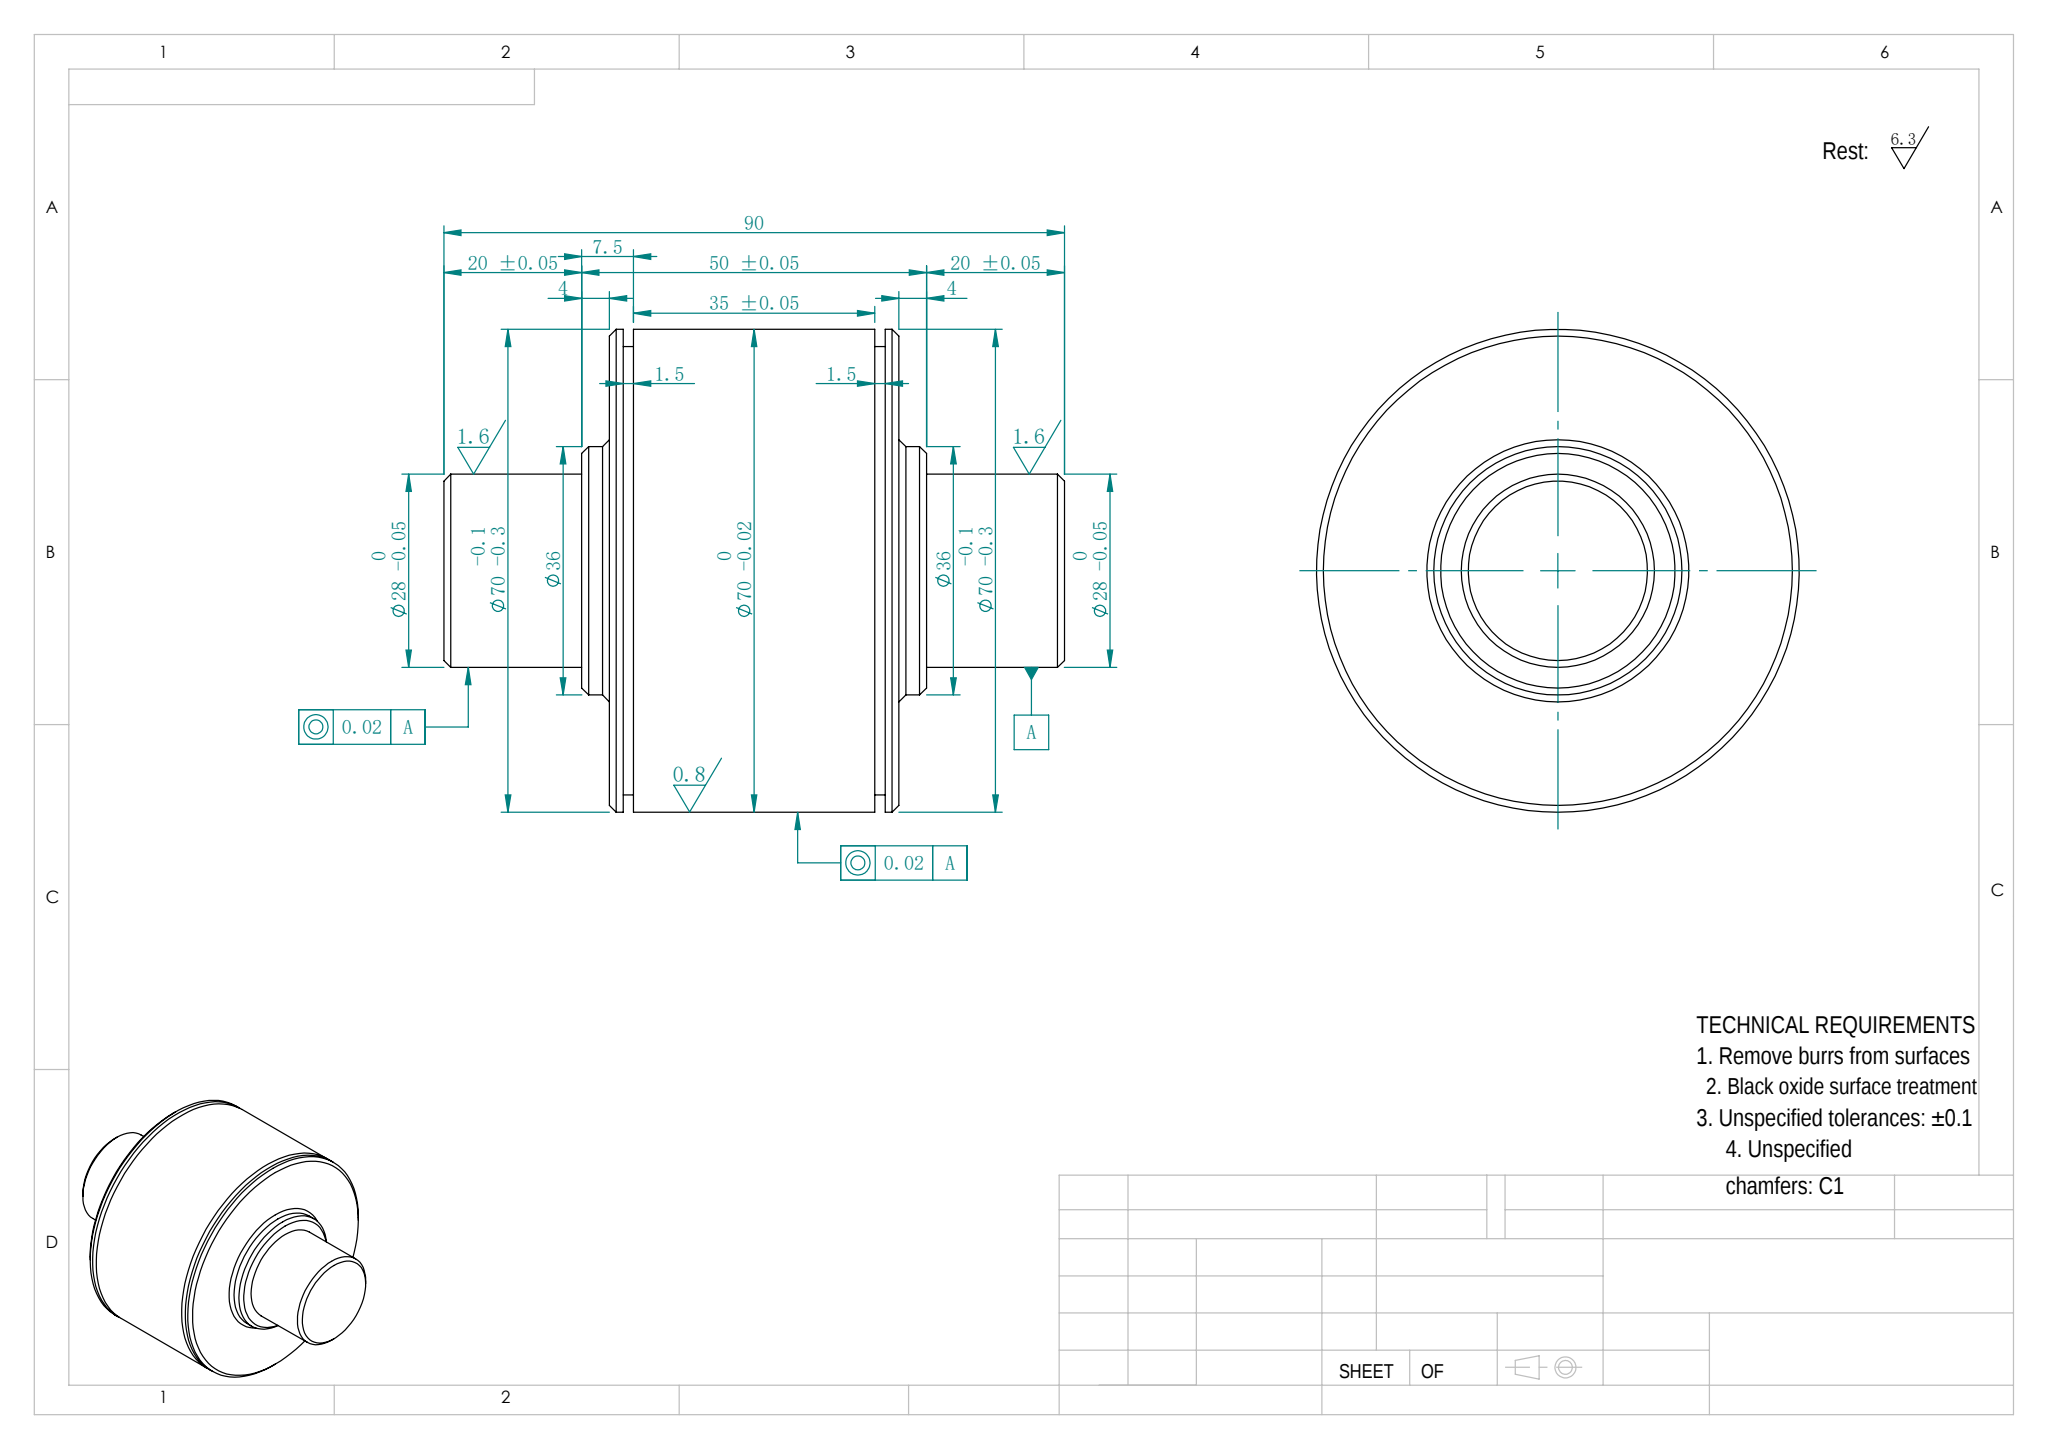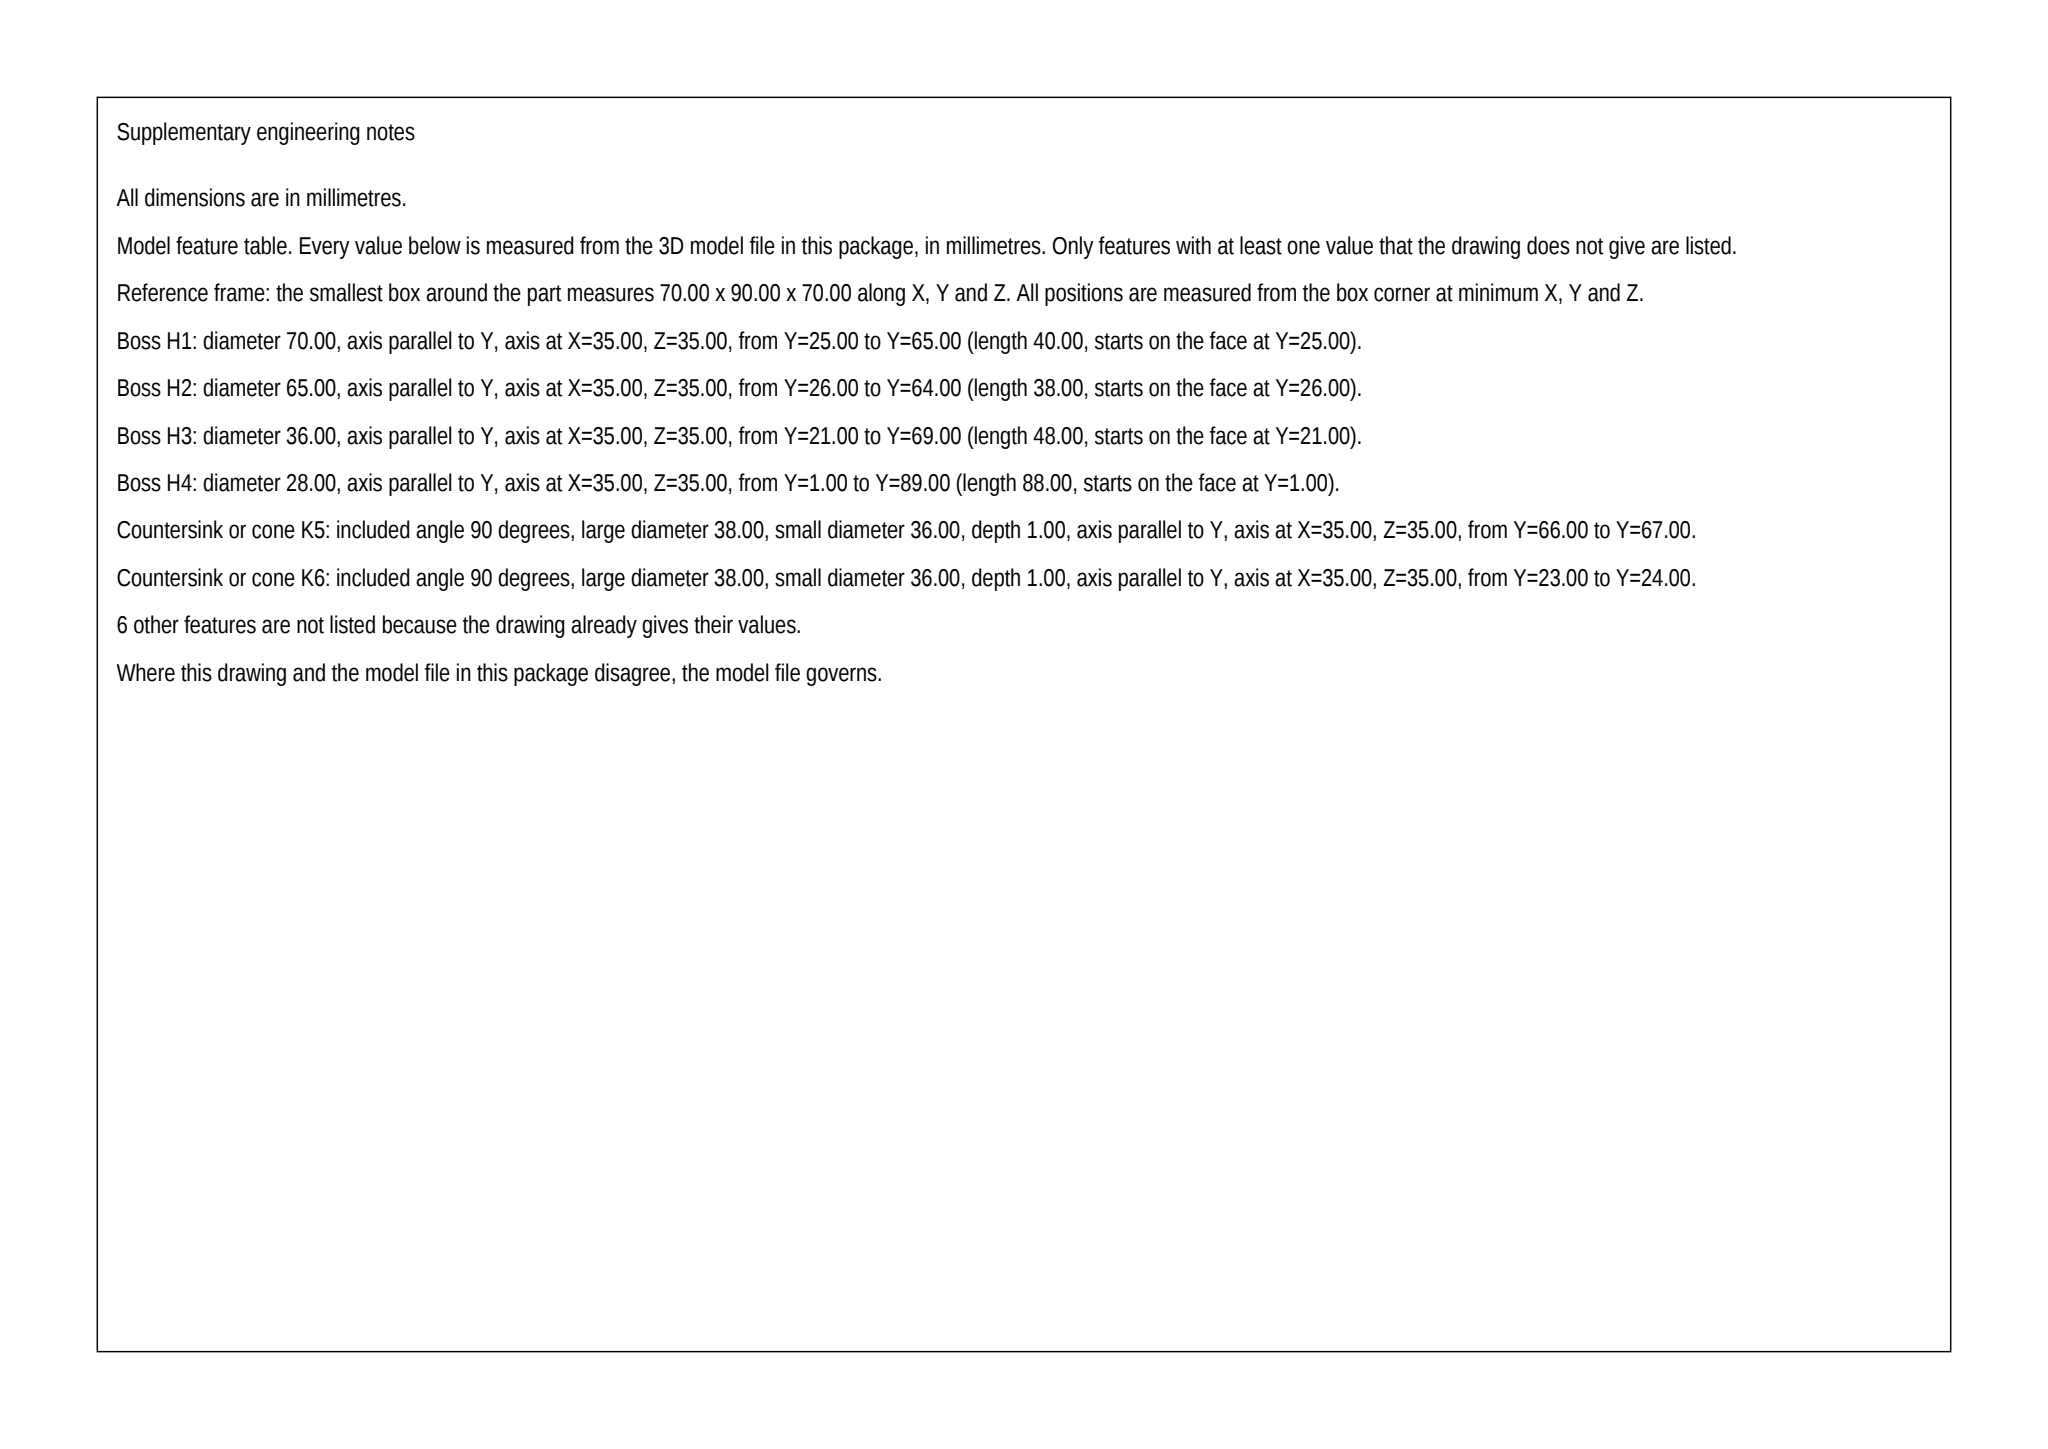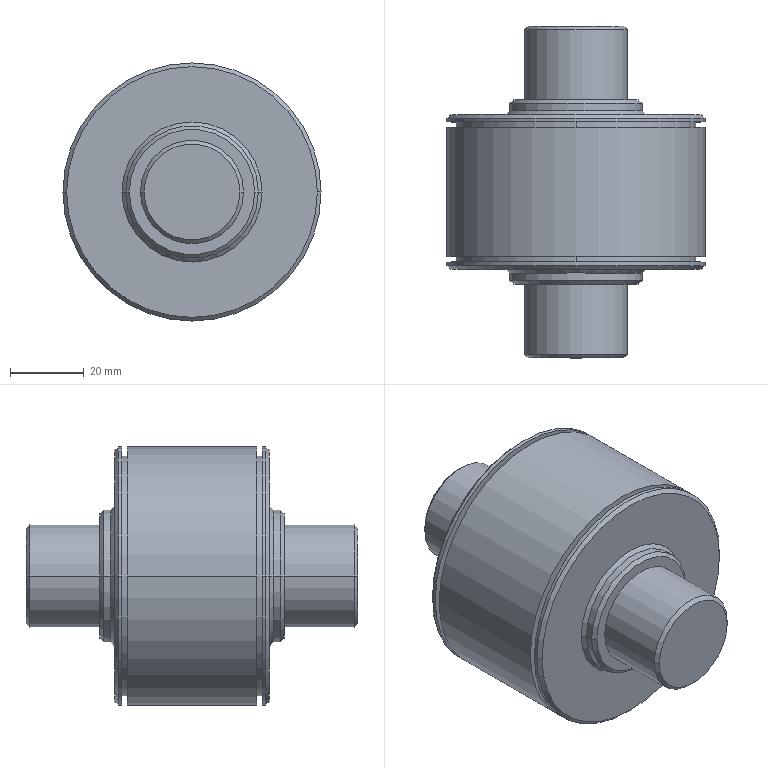Part | SolidWorks | mm | 1 solid | 44 faces | box 70 x 90 x 70 mm | volume 192518 mm3 | cylinder 18 | cone 16 | plane 10 | commonest cylinder face diameters 70 x6 36 x4 28 x4 65 x4
build123d program:
from build123d import *

# Parameters (mm, degrees)
SKETCH2_W     = 2.5
SKETCH2_H     = 1.5
CHAMFER1_SIZE = 1
CHAMFER2_SIZE = 1


with BuildPart() as part:
    # Sketch1 → Revolve1 (revolve)
    with BuildSketch(Plane.XY):
        Polygon((0, 0), (-14, 0), (-14, 20), (-18, 20), (-18, 24), (-35, 24), (-35, 66), (-18, 66), (-18, 70), (-14, 70), (-14, 90), (0, 90), align=None)
    revolve(axis=Axis((0, 90, 0), (0, -1, 0)))

    # Sketch2 → Cut-Revolve1 (revolve, cut)
    with BuildSketch(Plane.XY, mode=Mode.PRIVATE) as cut_revolve1_sk:
        with Locations((-33.75, 63.25)):
            Rectangle(SKETCH2_W, SKETCH2_H)
        with Locations((-33.75, 26.75)):
            Rectangle(SKETCH2_W, SKETCH2_H)
    revolve(cut_revolve1_sk.sketch.rotate(Axis((0, 0, 0), (0, 1, 0)), 270), axis=Axis((0, 0, 0), (0, 1, 0)), mode=Mode.SUBTRACT)

    # Chamfer1
    chamfer1_edges = [part.edges().sort_by_distance(p)[0] for p in [
        (35, 66, 0),
        (35, 24, 0),
        (18, 20, 0),
        (14, 0, 0),
        (14, 90, 0),
        (18, 70, 0),
    ]]
    chamfer(chamfer1_edges, length=CHAMFER1_SIZE)

    # Chamfer2
    chamfer2_edges = [part.edges().sort_by_distance(p)[0] for p in [
        (18, 66, 0),
        (18, 24, 0),
    ]]
    chamfer(chamfer2_edges, length=CHAMFER2_SIZE)


solid = part.part